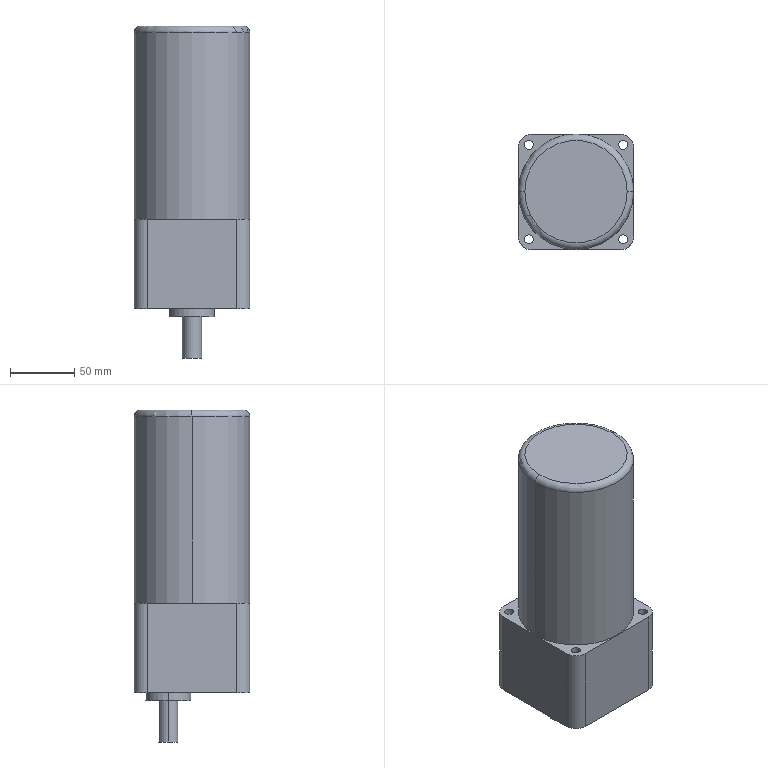Component | SolidWorks | JBM5120-502-01-2-1 | 1 solid | 29 faces | box 90 x 90 x 258.5 mm | volume 1509907 mm3 | cylinder 18 | plane 9 | torus 2 | commonest cylinder face diameters 7 x8 20 x4 15 x2 35 x2 89.8 x2
build123d program:
from build123d import *

# Parameters (mm, degrees)
SKETCH1_W          = 90
SKETCH1_H          = 90
EXTRUDE1_DEPTH     = 69.5
SKETCH2_R          = 44.9
EXTRUDE2_DEPTH     = 150.5
SKETCH3_R          = 3.5
CUT_EXTRUDE1_DEPTH = 230.02
SKETCH4_R          = 17.5
EXTRUDE3_DEPTH     = 6.5
SKETCH5_R          = 7.5
EXTRUDE4_DEPTH     = 32
FILLET1_R          = 10
FILLET2_R          = 5


with BuildPart() as part:
    # Sketch1 → Extrude1 (new body)
    with BuildSketch(Plane.XY):
        Rectangle(SKETCH1_W, SKETCH1_H)
    extrude(amount=-EXTRUDE1_DEPTH)

    # Sketch2 → Extrude2 (add)
    with BuildSketch(Plane(origin=(0, 0, -69.5), x_dir=(-1, 0, 0), z_dir=(0, 0, -1))):
        with Locations(Location((0, 0, 0), (0, 0, 180))):
            Circle(SKETCH2_R)
    extrude(amount=EXTRUDE2_DEPTH)

    # Sketch3 → Cut-Extrude1 (cut, through all)
    with BuildSketch(Plane.XY):
        with Locations((-36.75, 36.75)):
            Circle(SKETCH3_R)
        with Locations((36.75, 36.75)):
            Circle(SKETCH3_R)
        with Locations((36.75, -36.75)):
            Circle(SKETCH3_R)
        with Locations((-36.75, -36.75)):
            Circle(SKETCH3_R)
    extrude(amount=-CUT_EXTRUDE1_DEPTH, mode=Mode.SUBTRACT)

    # Sketch4 → Extrude3 (add)
    with BuildSketch(Plane.XY):
        with Locations(Location((0, 18.5, 0), (0, 0, 180))):
            Circle(SKETCH4_R)
    extrude(amount=EXTRUDE3_DEPTH)

    # Sketch5 → Extrude4 (add)
    with BuildSketch(Plane.XY.offset(6.5)):
        with Locations((0, 18.5)):
            Circle(SKETCH5_R)
    extrude(amount=EXTRUDE4_DEPTH)

    # Fillet1
    fillet1_edges = [part.edges().sort_by_distance(p)[0] for p in [
        (-45, 45, -34.75),
        (45, 45, -34.75),
        (45, -45, -34.75),
        (-45, -45, -34.75),
    ]]
    fillet(fillet1_edges, radius=FILLET1_R)

    # Fillet2
    fillet2_edges = [part.edges().sort_by_distance(p)[0] for p in [
        (-44.9, 0, -220),
    ]]
    fillet(fillet2_edges, radius=FILLET2_R)


solid = part.part

# Placed as in the assembly
solid = solid.moved(Location((647.283, -186.615, -151), (-180, 0, 180)))
STEP:
#1=COLOUR_RGB('',0.7922,0.8196,0.9333);
#2=FILL_AREA_STYLE_COLOUR('',#1);
#3=FILL_AREA_STYLE('',(#2));
#4=SURFACE_STYLE_FILL_AREA(#3);
#5=SURFACE_SIDE_STYLE('',(#4));
#6=SURFACE_STYLE_USAGE(.BOTH.,#5);
#7=PRESENTATION_STYLE_ASSIGNMENT((#6));
#8=CARTESIAN_POINT('',(23.716,-7.347,2.52));
#9=VERTEX_POINT('',#8);
#10=CARTESIAN_POINT('',(27.251,-7.347,2.52));
#11=VERTEX_POINT('',#10);
#12=CARTESIAN_POINT('',(25.484,-7.347,2.52));
#13=DIRECTION('',(0.,0.,-1.));
#14=DIRECTION('',(1.,0.,0.));
#15=AXIS2_PLACEMENT_3D('',#12,#13,#14);
#16=CIRCLE('',#15,1.768);
#17=EDGE_CURVE('',#9,#11,#16,.T.);
#18=ORIENTED_EDGE('',*,*,#17,.F.);
#19=CARTESIAN_POINT('',(23.913,-7.347,2.717));
#20=VERTEX_POINT('',#19);
#21=CARTESIAN_POINT('',(23.913,-7.347,2.52));
#22=DIRECTION('',(0.,1.,0.));
#23=DIRECTION('',(-1.,0.,0.));
#24=AXIS2_PLACEMENT_3D('',#21,#22,#23);
#25=CIRCLE('',#24,0.1969);
#26=EDGE_CURVE('',#9,#20,#25,.T.);
#27=ORIENTED_EDGE('',*,*,#26,.T.);
#28=CARTESIAN_POINT('',(27.054,-7.347,2.717));
#29=VERTEX_POINT('',#28);
#30=CARTESIAN_POINT('',(25.484,-7.347,2.717));
#31=DIRECTION('',(0.,0.,1.));
#32=DIRECTION('',(1.,0.,0.));
#33=AXIS2_PLACEMENT_3D('',#30,#31,#32);
#34=CIRCLE('',#33,1.571);
#35=EDGE_CURVE('',#29,#20,#34,.T.);
#36=ORIENTED_EDGE('',*,*,#35,.F.);
#37=CARTESIAN_POINT('',(27.054,-7.347,2.52));
#38=DIRECTION('',(-0.,-1.,0.));
#39=DIRECTION('',(1.,0.,0.));
#40=AXIS2_PLACEMENT_3D('',#37,#38,#39);
#41=CIRCLE('',#40,0.1969);
#42=EDGE_CURVE('',#11,#29,#41,.T.);
#43=ORIENTED_EDGE('',*,*,#42,.F.);
#44=EDGE_LOOP('',(#18,#27,#36,#43));
#45=FACE_OUTER_BOUND('',#44,.T.);
#46=CARTESIAN_POINT('',(25.484,-7.347,2.52));
#47=DIRECTION('',(0.,0.,1.));
#48=DIRECTION('',(1.,0.,0.));
#49=AXIS2_PLACEMENT_3D('',#46,#47,#48);
#50=TOROIDAL_SURFACE('',#49,1.571,0.1969);
#51=ADVANCED_FACE('',(#45),#50,.T.);
#52=CARTESIAN_POINT('',(25.188,-6.619,-7.461));
#53=VERTEX_POINT('',#52);
#54=CARTESIAN_POINT('',(25.779,-6.619,-7.461));
#55=VERTEX_POINT('',#54);
#56=CARTESIAN_POINT('',(25.484,-6.619,-7.461));
#57=DIRECTION('',(0.,0.,-1.));
#58=DIRECTION('',(-1.,0.,0.));
#59=AXIS2_PLACEMENT_3D('',#56,#57,#58);
#60=CIRCLE('',#59,0.2953);
#61=EDGE_CURVE('',#53,#55,#60,.T.);
#62=ORIENTED_EDGE('',*,*,#61,.F.);
#63=CARTESIAN_POINT('',(25.188,-6.619,-6.201));
#64=VERTEX_POINT('',#63);
#65=CARTESIAN_POINT('',(25.188,-6.619,-7.461));
#66=DIRECTION('',(0.,0.,1.));
#67=VECTOR('',#66,39.37);
#68=LINE('',#65,#67);
#69=EDGE_CURVE('',#53,#64,#68,.T.);
#70=ORIENTED_EDGE('',*,*,#69,.T.);
#71=CARTESIAN_POINT('',(25.779,-6.619,-6.201));
#72=VERTEX_POINT('',#71);
#73=CARTESIAN_POINT('',(25.484,-6.619,-6.201));
#74=DIRECTION('',(0.,0.,-1.));
#75=DIRECTION('',(-1.,0.,0.));
#76=AXIS2_PLACEMENT_3D('',#73,#74,#75);
#77=CIRCLE('',#76,0.2953);
#78=EDGE_CURVE('',#64,#72,#77,.T.);
#79=ORIENTED_EDGE('',*,*,#78,.T.);
#80=CARTESIAN_POINT('',(25.779,-6.619,-7.461));
#81=DIRECTION('',(0.,0.,1.));
#82=VECTOR('',#81,39.37);
#83=LINE('',#80,#82);
#84=EDGE_CURVE('',#55,#72,#83,.T.);
#85=ORIENTED_EDGE('',*,*,#84,.F.);
#86=EDGE_LOOP('',(#62,#70,#79,#85));
#87=FACE_OUTER_BOUND('',#86,.T.);
#88=CARTESIAN_POINT('',(25.484,-6.619,-7.461));
#89=DIRECTION('',(0.,0.,1.));
#90=DIRECTION('',(1.,0.,0.));
#91=AXIS2_PLACEMENT_3D('',#88,#89,#90);
#92=CYLINDRICAL_SURFACE('',#91,0.2953);
#93=ADVANCED_FACE('',(#87),#92,.T.);
#94=CARTESIAN_POINT('',(24.795,-6.619,-6.201));
#95=VERTEX_POINT('',#94);
#96=CARTESIAN_POINT('',(26.173,-6.619,-6.201));
#97=VERTEX_POINT('',#96);
#98=CARTESIAN_POINT('',(25.484,-6.619,-6.201));
#99=DIRECTION('',(0.,0.,-1.));
#100=DIRECTION('',(-1.,0.,0.));
#101=AXIS2_PLACEMENT_3D('',#98,#99,#100);
#102=CIRCLE('',#101,0.689);
#103=EDGE_CURVE('',#95,#97,#102,.T.);
#104=ORIENTED_EDGE('',*,*,#103,.F.);
#105=CARTESIAN_POINT('',(24.795,-6.619,-5.945));
#106=VERTEX_POINT('',#105);
#107=CARTESIAN_POINT('',(24.795,-6.619,-6.201));
#108=DIRECTION('',(0.,0.,1.));
#109=VECTOR('',#108,39.37);
#110=LINE('',#107,#109);
#111=EDGE_CURVE('',#95,#106,#110,.T.);
#112=ORIENTED_EDGE('',*,*,#111,.T.);
#113=CARTESIAN_POINT('',(26.173,-6.619,-5.945));
#114=VERTEX_POINT('',#113);
#115=CARTESIAN_POINT('',(25.484,-6.619,-5.945));
#116=DIRECTION('',(0.,0.,-1.));
#117=DIRECTION('',(-1.,0.,0.));
#118=AXIS2_PLACEMENT_3D('',#115,#116,#117);
#119=CIRCLE('',#118,0.689);
#120=EDGE_CURVE('',#106,#114,#119,.T.);
#121=ORIENTED_EDGE('',*,*,#120,.T.);
#122=CARTESIAN_POINT('',(26.173,-6.619,-6.201));
#123=DIRECTION('',(0.,0.,1.));
#124=VECTOR('',#123,39.37);
#125=LINE('',#122,#124);
#126=EDGE_CURVE('',#97,#114,#125,.T.);
#127=ORIENTED_EDGE('',*,*,#126,.F.);
#128=EDGE_LOOP('',(#104,#112,#121,#127));
#129=FACE_OUTER_BOUND('',#128,.T.);
#130=CARTESIAN_POINT('',(25.484,-6.619,-6.201));
#131=DIRECTION('',(0.,0.,1.));
#132=DIRECTION('',(1.,0.,0.));
#133=AXIS2_PLACEMENT_3D('',#130,#131,#132);
#134=CYLINDRICAL_SURFACE('',#133,0.689);
#135=ADVANCED_FACE('',(#129),#134,.T.);
#136=CARTESIAN_POINT('',(27.068,-8.794,-3.209));
#137=VERTEX_POINT('',#136);
#138=CARTESIAN_POINT('',(26.793,-8.794,-3.209));
#139=VERTEX_POINT('',#138);
#140=CARTESIAN_POINT('',(26.93,-8.794,-3.209));
#141=DIRECTION('',(0.,0.,-1.));
#142=DIRECTION('',(-1.,0.,0.));
#143=AXIS2_PLACEMENT_3D('',#140,#141,#142);
#144=CIRCLE('',#143,0.1378);
#145=EDGE_CURVE('',#137,#139,#144,.T.);
#146=ORIENTED_EDGE('',*,*,#145,.F.);
#147=CARTESIAN_POINT('',(27.068,-8.794,-5.945));
#148=VERTEX_POINT('',#147);
#149=CARTESIAN_POINT('',(27.068,-8.794,2.717));
#150=DIRECTION('',(0.,0.,-1.));
#151=VECTOR('',#150,39.37);
#152=LINE('',#149,#151);
#153=EDGE_CURVE('',#137,#148,#152,.T.);
#154=ORIENTED_EDGE('',*,*,#153,.T.);
#155=CARTESIAN_POINT('',(26.793,-8.794,-5.945));
#156=VERTEX_POINT('',#155);
#157=CARTESIAN_POINT('',(26.93,-8.794,-5.945));
#158=DIRECTION('',(0.,0.,-1.));
#159=DIRECTION('',(1.,0.,0.));
#160=AXIS2_PLACEMENT_3D('',#157,#158,#159);
#161=CIRCLE('',#160,0.1378);
#162=EDGE_CURVE('',#148,#156,#161,.T.);
#163=ORIENTED_EDGE('',*,*,#162,.T.);
#164=CARTESIAN_POINT('',(26.793,-8.794,2.717));
#165=DIRECTION('',(0.,0.,-1.));
#166=VECTOR('',#165,39.37);
#167=LINE('',#164,#166);
#168=EDGE_CURVE('',#139,#156,#167,.T.);
#169=ORIENTED_EDGE('',*,*,#168,.F.);
#170=EDGE_LOOP('',(#146,#154,#163,#169));
#171=FACE_OUTER_BOUND('',#170,.T.);
#172=CARTESIAN_POINT('',(26.93,-8.794,2.717));
#173=DIRECTION('',(0.,0.,-1.));
#174=DIRECTION('',(-1.,0.,0.));
#175=AXIS2_PLACEMENT_3D('',#172,#173,#174);
#176=CYLINDRICAL_SURFACE('',#175,0.1378);
#177=ADVANCED_FACE('',(#171),#176,.F.);
#178=CARTESIAN_POINT('',(24.175,-8.794,-3.209));
#179=VERTEX_POINT('',#178);
#180=CARTESIAN_POINT('',(23.899,-8.794,-3.209));
#181=VERTEX_POINT('',#180);
#182=CARTESIAN_POINT('',(24.037,-8.794,-3.209));
#183=DIRECTION('',(0.,0.,-1.));
#184=DIRECTION('',(-1.,0.,0.));
#185=AXIS2_PLACEMENT_3D('',#182,#183,#184);
#186=CIRCLE('',#185,0.1378);
#187=EDGE_CURVE('',#179,#181,#186,.T.);
#188=ORIENTED_EDGE('',*,*,#187,.F.);
#189=CARTESIAN_POINT('',(24.175,-8.794,-5.945));
#190=VERTEX_POINT('',#189);
#191=CARTESIAN_POINT('',(24.175,-8.794,2.717));
#192=DIRECTION('',(0.,0.,-1.));
#193=VECTOR('',#192,39.37);
#194=LINE('',#191,#193);
#195=EDGE_CURVE('',#179,#190,#194,.T.);
#196=ORIENTED_EDGE('',*,*,#195,.T.);
#197=CARTESIAN_POINT('',(23.899,-8.794,-5.945));
#198=VERTEX_POINT('',#197);
#199=CARTESIAN_POINT('',(24.037,-8.794,-5.945));
#200=DIRECTION('',(0.,0.,-1.));
#201=DIRECTION('',(-1.,0.,0.));
#202=AXIS2_PLACEMENT_3D('',#199,#200,#201);
#203=CIRCLE('',#202,0.1378);
#204=EDGE_CURVE('',#190,#198,#203,.T.);
#205=ORIENTED_EDGE('',*,*,#204,.T.);
#206=CARTESIAN_POINT('',(23.899,-8.794,2.717));
#207=DIRECTION('',(0.,0.,-1.));
#208=VECTOR('',#207,39.37);
#209=LINE('',#206,#208);
#210=EDGE_CURVE('',#181,#198,#209,.T.);
#211=ORIENTED_EDGE('',*,*,#210,.F.);
#212=EDGE_LOOP('',(#188,#196,#205,#211));
#213=FACE_OUTER_BOUND('',#212,.T.);
#214=CARTESIAN_POINT('',(24.037,-8.794,2.717));
#215=DIRECTION('',(0.,0.,-1.));
#216=DIRECTION('',(-1.,0.,0.));
#217=AXIS2_PLACEMENT_3D('',#214,#215,#216);
#218=CYLINDRICAL_SURFACE('',#217,0.1378);
#219=ADVANCED_FACE('',(#213),#218,.F.);
#220=CARTESIAN_POINT('',(24.175,-5.9,-3.209));
#221=VERTEX_POINT('',#220);
#222=CARTESIAN_POINT('',(23.899,-5.9,-3.209));
#223=VERTEX_POINT('',#222);
#224=CARTESIAN_POINT('',(24.037,-5.9,-3.209));
#225=DIRECTION('',(0.,0.,-1.));
#226=DIRECTION('',(-1.,0.,0.));
#227=AXIS2_PLACEMENT_3D('',#224,#225,#226);
#228=CIRCLE('',#227,0.1378);
#229=EDGE_CURVE('',#221,#223,#228,.T.);
#230=ORIENTED_EDGE('',*,*,#229,.F.);
#231=CARTESIAN_POINT('',(24.175,-5.9,-5.945));
#232=VERTEX_POINT('',#231);
#233=CARTESIAN_POINT('',(24.175,-5.9,2.717));
#234=DIRECTION('',(0.,0.,-1.));
#235=VECTOR('',#234,39.37);
#236=LINE('',#233,#235);
#237=EDGE_CURVE('',#221,#232,#236,.T.);
#238=ORIENTED_EDGE('',*,*,#237,.T.);
#239=CARTESIAN_POINT('',(23.899,-5.9,-5.945));
#240=VERTEX_POINT('',#239);
#241=CARTESIAN_POINT('',(24.037,-5.9,-5.945));
#242=DIRECTION('',(0.,0.,-1.));
#243=DIRECTION('',(1.,0.,0.));
#244=AXIS2_PLACEMENT_3D('',#241,#242,#243);
#245=CIRCLE('',#244,0.1378);
#246=EDGE_CURVE('',#232,#240,#245,.T.);
#247=ORIENTED_EDGE('',*,*,#246,.T.);
#248=CARTESIAN_POINT('',(23.899,-5.9,2.717));
#249=DIRECTION('',(0.,0.,-1.));
#250=VECTOR('',#249,39.37);
#251=LINE('',#248,#250);
#252=EDGE_CURVE('',#223,#240,#251,.T.);
#253=ORIENTED_EDGE('',*,*,#252,.F.);
#254=EDGE_LOOP('',(#230,#238,#247,#253));
#255=FACE_OUTER_BOUND('',#254,.T.);
#256=CARTESIAN_POINT('',(24.037,-5.9,2.717));
#257=DIRECTION('',(0.,0.,-1.));
#258=DIRECTION('',(-1.,0.,0.));
#259=AXIS2_PLACEMENT_3D('',#256,#257,#258);
#260=CYLINDRICAL_SURFACE('',#259,0.1378);
#261=ADVANCED_FACE('',(#255),#260,.F.);
#262=CARTESIAN_POINT('',(27.068,-5.9,-3.209));
#263=VERTEX_POINT('',#262);
#264=CARTESIAN_POINT('',(26.793,-5.9,-3.209));
#265=VERTEX_POINT('',#264);
#266=CARTESIAN_POINT('',(26.93,-5.9,-3.209));
#267=DIRECTION('',(0.,0.,-1.));
#268=DIRECTION('',(-1.,0.,0.));
#269=AXIS2_PLACEMENT_3D('',#266,#267,#268);
#270=CIRCLE('',#269,0.1378);
#271=EDGE_CURVE('',#263,#265,#270,.T.);
#272=ORIENTED_EDGE('',*,*,#271,.F.);
#273=CARTESIAN_POINT('',(27.068,-5.9,-5.945));
#274=VERTEX_POINT('',#273);
#275=CARTESIAN_POINT('',(27.068,-5.9,2.717));
#276=DIRECTION('',(0.,0.,-1.));
#277=VECTOR('',#276,39.37);
#278=LINE('',#275,#277);
#279=EDGE_CURVE('',#263,#274,#278,.T.);
#280=ORIENTED_EDGE('',*,*,#279,.T.);
#281=CARTESIAN_POINT('',(26.793,-5.9,-5.945));
#282=VERTEX_POINT('',#281);
#283=CARTESIAN_POINT('',(26.93,-5.9,-5.945));
#284=DIRECTION('',(0.,0.,-1.));
#285=DIRECTION('',(-1.,0.,0.));
#286=AXIS2_PLACEMENT_3D('',#283,#284,#285);
#287=CIRCLE('',#286,0.1378);
#288=EDGE_CURVE('',#274,#282,#287,.T.);
#289=ORIENTED_EDGE('',*,*,#288,.T.);
#290=CARTESIAN_POINT('',(26.793,-5.9,2.717));
#291=DIRECTION('',(0.,0.,-1.));
#292=VECTOR('',#291,39.37);
#293=LINE('',#290,#292);
#294=EDGE_CURVE('',#265,#282,#293,.T.);
#295=ORIENTED_EDGE('',*,*,#294,.F.);
#296=EDGE_LOOP('',(#272,#280,#289,#295));
#297=FACE_OUTER_BOUND('',#296,.T.);
#298=CARTESIAN_POINT('',(26.93,-5.9,2.717));
#299=DIRECTION('',(0.,0.,-1.));
#300=DIRECTION('',(-1.,0.,0.));
#301=AXIS2_PLACEMENT_3D('',#298,#299,#300);
#302=CYLINDRICAL_SURFACE('',#301,0.1378);
#303=ADVANCED_FACE('',(#297),#302,.F.);
#304=ORIENTED_EDGE('',*,*,#17,.T.);
#305=CARTESIAN_POINT('',(27.251,-7.347,-3.209));
#306=VERTEX_POINT('',#305);
#307=CARTESIAN_POINT('',(27.251,-7.347,2.717));
#308=DIRECTION('',(0.,0.,-1.));
#309=VECTOR('',#308,39.37);
#310=LINE('',#307,#309);
#311=EDGE_CURVE('',#11,#306,#310,.T.);
#312=ORIENTED_EDGE('',*,*,#311,.T.);
#313=CARTESIAN_POINT('',(23.716,-7.347,-3.209));
#314=VERTEX_POINT('',#313);
#315=CARTESIAN_POINT('',(25.484,-7.347,-3.209));
#316=DIRECTION('',(0.,0.,1.));
#317=DIRECTION('',(-1.,0.,0.));
#318=AXIS2_PLACEMENT_3D('',#315,#316,#317);
#319=CIRCLE('',#318,1.768);
#320=EDGE_CURVE('',#306,#314,#319,.T.);
#321=ORIENTED_EDGE('',*,*,#320,.T.);
#322=CARTESIAN_POINT('',(23.716,-7.347,2.717));
#323=DIRECTION('',(0.,0.,-1.));
#324=VECTOR('',#323,39.37);
#325=LINE('',#322,#324);
#326=EDGE_CURVE('',#9,#314,#325,.T.);
#327=ORIENTED_EDGE('',*,*,#326,.F.);
#328=EDGE_LOOP('',(#304,#312,#321,#327));
#329=FACE_OUTER_BOUND('',#328,.T.);
#330=CARTESIAN_POINT('',(25.484,-7.347,2.717));
#331=DIRECTION('',(0.,0.,-1.));
#332=DIRECTION('',(-1.,0.,0.));
#333=AXIS2_PLACEMENT_3D('',#330,#331,#332);
#334=CYLINDRICAL_SURFACE('',#333,1.768);
#335=ADVANCED_FACE('',(#329),#334,.T.);
#336=CARTESIAN_POINT('',(25.484,-6.619,-6.201));
#337=DIRECTION('',(0.,0.,-1.));
#338=DIRECTION('',(-1.,0.,0.));
#339=AXIS2_PLACEMENT_3D('',#336,#337,#338);
#340=CIRCLE('',#339,0.689);
#341=EDGE_CURVE('',#97,#95,#340,.T.);
#342=ORIENTED_EDGE('',*,*,#341,.T.);
#343=ORIENTED_EDGE('',*,*,#103,.T.);
#344=EDGE_LOOP('',(#342,#343));
#345=FACE_OUTER_BOUND('',#344,.T.);
#346=CARTESIAN_POINT('',(25.484,-6.619,-6.201));
#347=DIRECTION('',(0.,0.,-1.));
#348=DIRECTION('',(-1.,0.,0.));
#349=AXIS2_PLACEMENT_3D('',#346,#347,#348);
#350=CIRCLE('',#349,0.2953);
#351=EDGE_CURVE('',#72,#64,#350,.T.);
#352=ORIENTED_EDGE('',*,*,#351,.F.);
#353=ORIENTED_EDGE('',*,*,#78,.F.);
#354=EDGE_LOOP('',(#352,#353));
#355=FACE_BOUND('',#354,.T.);
#356=CARTESIAN_POINT('',(25.484,-6.619,-6.201));
#357=DIRECTION('',(0.,0.,-1.));
#358=DIRECTION('',(-1.,0.,0.));
#359=AXIS2_PLACEMENT_3D('',#356,#357,#358);
#360=PLANE('',#359);
#361=ADVANCED_FACE('',(#345,#355),#360,.T.);
#362=CARTESIAN_POINT('',(27.255,-5.969,-5.945));
#363=VERTEX_POINT('',#362);
#364=CARTESIAN_POINT('',(27.255,-8.725,-5.945));
#365=VERTEX_POINT('',#364);
#366=CARTESIAN_POINT('',(27.255,-5.575,-5.945));
#367=DIRECTION('',(-0.,-1.,0.));
#368=VECTOR('',#367,39.37);
#369=LINE('',#366,#368);
#370=EDGE_CURVE('',#363,#365,#369,.T.);
#371=ORIENTED_EDGE('',*,*,#370,.T.);
#372=CARTESIAN_POINT('',(26.862,-9.119,-5.945));
#373=VERTEX_POINT('',#372);
#374=CARTESIAN_POINT('',(26.862,-8.725,-5.945));
#375=DIRECTION('',(0.,0.,-1.));
#376=DIRECTION('',(-1.,0.,0.));
#377=AXIS2_PLACEMENT_3D('',#374,#375,#376);
#378=CIRCLE('',#377,0.3937);
#379=EDGE_CURVE('',#365,#373,#378,.T.);
#380=ORIENTED_EDGE('',*,*,#379,.T.);
#381=CARTESIAN_POINT('',(24.106,-9.119,-5.945));
#382=VERTEX_POINT('',#381);
#383=CARTESIAN_POINT('',(27.255,-9.119,-5.945));
#384=DIRECTION('',(-1.,0.,0.));
#385=VECTOR('',#384,39.37);
#386=LINE('',#383,#385);
#387=EDGE_CURVE('',#373,#382,#386,.T.);
#388=ORIENTED_EDGE('',*,*,#387,.T.);
#389=CARTESIAN_POINT('',(23.712,-8.725,-5.945));
#390=VERTEX_POINT('',#389);
#391=CARTESIAN_POINT('',(24.106,-8.725,-5.945));
#392=DIRECTION('',(0.,0.,-1.));
#393=DIRECTION('',(-1.,0.,0.));
#394=AXIS2_PLACEMENT_3D('',#391,#392,#393);
#395=CIRCLE('',#394,0.3937);
#396=EDGE_CURVE('',#382,#390,#395,.T.);
#397=ORIENTED_EDGE('',*,*,#396,.T.);
#398=CARTESIAN_POINT('',(23.712,-5.969,-5.945));
#399=VERTEX_POINT('',#398);
#400=CARTESIAN_POINT('',(23.712,-5.575,-5.945));
#401=DIRECTION('',(0.,1.,0.));
#402=VECTOR('',#401,39.37);
#403=LINE('',#400,#402);
#404=EDGE_CURVE('',#390,#399,#403,.T.);
#405=ORIENTED_EDGE('',*,*,#404,.T.);
#406=CARTESIAN_POINT('',(24.106,-5.575,-5.945));
#407=VERTEX_POINT('',#406);
#408=CARTESIAN_POINT('',(24.106,-5.969,-5.945));
#409=DIRECTION('',(0.,0.,-1.));
#410=DIRECTION('',(-1.,0.,0.));
#411=AXIS2_PLACEMENT_3D('',#408,#409,#410);
#412=CIRCLE('',#411,0.3937);
#413=EDGE_CURVE('',#399,#407,#412,.T.);
#414=ORIENTED_EDGE('',*,*,#413,.T.);
#415=CARTESIAN_POINT('',(26.862,-5.575,-5.945));
#416=VERTEX_POINT('',#415);
#417=CARTESIAN_POINT('',(27.255,-5.575,-5.945));
#418=DIRECTION('',(1.,-0.,0.));
#419=VECTOR('',#418,39.37);
#420=LINE('',#417,#419);
#421=EDGE_CURVE('',#407,#416,#420,.T.);
#422=ORIENTED_EDGE('',*,*,#421,.T.);
#423=CARTESIAN_POINT('',(26.862,-5.969,-5.945));
#424=DIRECTION('',(0.,0.,-1.));
#425=DIRECTION('',(-1.,0.,0.));
#426=AXIS2_PLACEMENT_3D('',#423,#424,#425);
#427=CIRCLE('',#426,0.3937);
#428=EDGE_CURVE('',#416,#363,#427,.T.);
#429=ORIENTED_EDGE('',*,*,#428,.T.);
#430=EDGE_LOOP('',(#371,#380,#388,#397,#405,#414,#422,#429));
#431=FACE_OUTER_BOUND('',#430,.T.);
#432=CARTESIAN_POINT('',(26.93,-5.9,-5.945));
#433=DIRECTION('',(0.,0.,-1.));
#434=DIRECTION('',(-1.,0.,0.));
#435=AXIS2_PLACEMENT_3D('',#432,#433,#434);
#436=CIRCLE('',#435,0.1378);
#437=EDGE_CURVE('',#282,#274,#436,.T.);
#438=ORIENTED_EDGE('',*,*,#437,.F.);
#439=ORIENTED_EDGE('',*,*,#288,.F.);
#440=EDGE_LOOP('',(#438,#439));
#441=FACE_BOUND('',#440,.T.);
#442=CARTESIAN_POINT('',(24.037,-5.9,-5.945));
#443=DIRECTION('',(0.,0.,-1.));
#444=DIRECTION('',(1.,0.,0.));
#445=AXIS2_PLACEMENT_3D('',#442,#443,#444);
#446=CIRCLE('',#445,0.1378);
#447=EDGE_CURVE('',#240,#232,#446,.T.);
#448=ORIENTED_EDGE('',*,*,#447,.F.);
#449=ORIENTED_EDGE('',*,*,#246,.F.);
#450=EDGE_LOOP('',(#448,#449));
#451=FACE_BOUND('',#450,.T.);
#452=CARTESIAN_POINT('',(24.037,-8.794,-5.945));
#453=DIRECTION('',(0.,0.,-1.));
#454=DIRECTION('',(-1.,0.,0.));
#455=AXIS2_PLACEMENT_3D('',#452,#453,#454);
#456=CIRCLE('',#455,0.1378);
#457=EDGE_CURVE('',#198,#190,#456,.T.);
#458=ORIENTED_EDGE('',*,*,#457,.F.);
#459=ORIENTED_EDGE('',*,*,#204,.F.);
#460=EDGE_LOOP('',(#458,#459));
#461=FACE_BOUND('',#460,.T.);
#462=CARTESIAN_POINT('',(26.93,-8.794,-5.945));
#463=DIRECTION('',(0.,0.,-1.));
#464=DIRECTION('',(1.,0.,0.));
#465=AXIS2_PLACEMENT_3D('',#462,#463,#464);
#466=CIRCLE('',#465,0.1378);
#467=EDGE_CURVE('',#156,#148,#466,.T.);
#468=ORIENTED_EDGE('',*,*,#467,.F.);
#469=ORIENTED_EDGE('',*,*,#162,.F.);
#470=EDGE_LOOP('',(#468,#469));
#471=FACE_BOUND('',#470,.T.);
#472=CARTESIAN_POINT('',(25.484,-6.619,-5.945));
#473=DIRECTION('',(0.,0.,-1.));
#474=DIRECTION('',(-1.,0.,0.));
#475=AXIS2_PLACEMENT_3D('',#472,#473,#474);
#476=CIRCLE('',#475,0.689);
#477=EDGE_CURVE('',#114,#106,#476,.T.);
#478=ORIENTED_EDGE('',*,*,#477,.F.);
#479=ORIENTED_EDGE('',*,*,#120,.F.);
#480=EDGE_LOOP('',(#478,#479));
#481=FACE_BOUND('',#480,.T.);
#482=CARTESIAN_POINT('',(27.255,-9.119,-5.945));
#483=DIRECTION('',(0.,0.,-1.));
#484=DIRECTION('',(-1.,0.,0.));
#485=AXIS2_PLACEMENT_3D('',#482,#483,#484);
#486=PLANE('',#485);
#487=ADVANCED_FACE('',(#431,#441,#451,#461,#471,#481),#486,.T.);
#488=CARTESIAN_POINT('',(26.93,-8.794,-3.209));
#489=DIRECTION('',(0.,0.,-1.));
#490=DIRECTION('',(-1.,0.,0.));
#491=AXIS2_PLACEMENT_3D('',#488,#489,#490);
#492=CIRCLE('',#491,0.1378);
#493=EDGE_CURVE('',#139,#137,#492,.T.);
#494=ORIENTED_EDGE('',*,*,#493,.T.);
#495=ORIENTED_EDGE('',*,*,#145,.T.);
#496=EDGE_LOOP('',(#494,#495));
#497=FACE_BOUND('',#496,.T.);
#498=CARTESIAN_POINT('',(24.037,-8.794,-3.209));
#499=DIRECTION('',(0.,0.,-1.));
#500=DIRECTION('',(-1.,0.,0.));
#501=AXIS2_PLACEMENT_3D('',#498,#499,#500);
#502=CIRCLE('',#501,0.1378);
#503=EDGE_CURVE('',#181,#179,#502,.T.);
#504=ORIENTED_EDGE('',*,*,#503,.T.);
#505=ORIENTED_EDGE('',*,*,#187,.T.);
#506=EDGE_LOOP('',(#504,#505));
#507=FACE_BOUND('',#506,.T.);
#508=CARTESIAN_POINT('',(24.037,-5.9,-3.209));
#509=DIRECTION('',(0.,0.,-1.));
#510=DIRECTION('',(-1.,0.,0.));
#511=AXIS2_PLACEMENT_3D('',#508,#509,#510);
#512=CIRCLE('',#511,0.1378);
#513=EDGE_CURVE('',#223,#221,#512,.T.);
#514=ORIENTED_EDGE('',*,*,#513,.T.);
#515=ORIENTED_EDGE('',*,*,#229,.T.);
#516=EDGE_LOOP('',(#514,#515));
#517=FACE_BOUND('',#516,.T.);
#518=CARTESIAN_POINT('',(26.93,-5.9,-3.209));
#519=DIRECTION('',(0.,0.,-1.));
#520=DIRECTION('',(-1.,0.,0.));
#521=AXIS2_PLACEMENT_3D('',#518,#519,#520);
#522=CIRCLE('',#521,0.1378);
#523=EDGE_CURVE('',#265,#263,#522,.T.);
#524=ORIENTED_EDGE('',*,*,#523,.T.);
#525=ORIENTED_EDGE('',*,*,#271,.T.);
#526=EDGE_LOOP('',(#524,#525));
#527=FACE_BOUND('',#526,.T.);
#528=CARTESIAN_POINT('',(26.862,-9.119,-3.209));
#529=VERTEX_POINT('',#528);
#530=CARTESIAN_POINT('',(24.106,-9.119,-3.209));
#531=VERTEX_POINT('',#530);
#532=CARTESIAN_POINT('',(27.255,-9.119,-3.209));
#533=DIRECTION('',(-1.,0.,0.));
#534=VECTOR('',#533,39.37);
#535=LINE('',#532,#534);
#536=EDGE_CURVE('',#529,#531,#535,.T.);
#537=ORIENTED_EDGE('',*,*,#536,.F.);
#538=CARTESIAN_POINT('',(27.255,-8.725,-3.209));
#539=VERTEX_POINT('',#538);
#540=CARTESIAN_POINT('',(26.862,-8.725,-3.209));
#541=DIRECTION('',(0.,0.,1.));
#542=DIRECTION('',(-1.,0.,0.));
#543=AXIS2_PLACEMENT_3D('',#540,#541,#542);
#544=CIRCLE('',#543,0.3937);
#545=EDGE_CURVE('',#529,#539,#544,.T.);
#546=ORIENTED_EDGE('',*,*,#545,.T.);
#547=CARTESIAN_POINT('',(27.255,-5.969,-3.209));
#548=VERTEX_POINT('',#547);
#549=CARTESIAN_POINT('',(27.255,-5.575,-3.209));
#550=DIRECTION('',(-0.,-1.,0.));
#551=VECTOR('',#550,39.37);
#552=LINE('',#549,#551);
#553=EDGE_CURVE('',#548,#539,#552,.T.);
#554=ORIENTED_EDGE('',*,*,#553,.F.);
#555=CARTESIAN_POINT('',(26.862,-5.575,-3.209));
#556=VERTEX_POINT('',#555);
#557=CARTESIAN_POINT('',(26.862,-5.969,-3.209));
#558=DIRECTION('',(0.,0.,1.));
#559=DIRECTION('',(-1.,0.,0.));
#560=AXIS2_PLACEMENT_3D('',#557,#558,#559);
#561=CIRCLE('',#560,0.3937);
#562=EDGE_CURVE('',#548,#556,#561,.T.);
#563=ORIENTED_EDGE('',*,*,#562,.T.);
#564=CARTESIAN_POINT('',(24.106,-5.575,-3.209));
#565=VERTEX_POINT('',#564);
#566=CARTESIAN_POINT('',(27.255,-5.575,-3.209));
#567=DIRECTION('',(1.,-0.,0.));
#568=VECTOR('',#567,39.37);
#569=LINE('',#566,#568);
#570=EDGE_CURVE('',#565,#556,#569,.T.);
#571=ORIENTED_EDGE('',*,*,#570,.F.);
#572=CARTESIAN_POINT('',(23.712,-5.969,-3.209));
#573=VERTEX_POINT('',#572);
#574=CARTESIAN_POINT('',(24.106,-5.969,-3.209));
#575=DIRECTION('',(0.,0.,1.));
#576=DIRECTION('',(-1.,-0.,0.));
#577=AXIS2_PLACEMENT_3D('',#574,#575,#576);
#578=CIRCLE('',#577,0.3937);
#579=EDGE_CURVE('',#565,#573,#578,.T.);
#580=ORIENTED_EDGE('',*,*,#579,.T.);
#581=CARTESIAN_POINT('',(23.712,-8.725,-3.209));
#582=VERTEX_POINT('',#581);
#583=CARTESIAN_POINT('',(23.712,-5.575,-3.209));
#584=DIRECTION('',(0.,1.,0.));
#585=VECTOR('',#584,39.37);
#586=LINE('',#583,#585);
#587=EDGE_CURVE('',#582,#573,#586,.T.);
#588=ORIENTED_EDGE('',*,*,#587,.F.);
#589=CARTESIAN_POINT('',(24.106,-8.725,-3.209));
#590=DIRECTION('',(0.,0.,1.));
#591=DIRECTION('',(-1.,0.,0.));
#592=AXIS2_PLACEMENT_3D('',#589,#590,#591);
#593=CIRCLE('',#592,0.3937);
#594=EDGE_CURVE('',#582,#531,#593,.T.);
#595=ORIENTED_EDGE('',*,*,#594,.T.);
#596=EDGE_LOOP('',(#537,#546,#554,#563,#571,#580,#588,#595));
#597=FACE_OUTER_BOUND('',#596,.T.);
#598=CARTESIAN_POINT('',(25.484,-7.347,-3.209));
#599=DIRECTION('',(0.,0.,1.));
#600=DIRECTION('',(-1.,0.,0.));
#601=AXIS2_PLACEMENT_3D('',#598,#599,#600);
#602=CIRCLE('',#601,1.768);
#603=EDGE_CURVE('',#314,#306,#602,.T.);
#604=ORIENTED_EDGE('',*,*,#603,.F.);
#605=ORIENTED_EDGE('',*,*,#320,.F.);
#606=EDGE_LOOP('',(#604,#605));
#607=FACE_BOUND('',#606,.T.);
#608=CARTESIAN_POINT('',(27.255,-9.119,-3.209));
#609=DIRECTION('',(0.,0.,-1.));
#610=DIRECTION('',(-1.,0.,0.));
#611=AXIS2_PLACEMENT_3D('',#608,#609,#610);
#612=PLANE('',#611);
#613=ADVANCED_FACE('',(#497,#507,#517,#527,#597,#607),#612,.F.);
#614=ORIENTED_EDGE('',*,*,#553,.T.);
#615=CARTESIAN_POINT('',(27.255,-8.725,-3.209));
#616=DIRECTION('',(0.,0.,-1.));
#617=VECTOR('',#616,39.37);
#618=LINE('',#615,#617);
#619=EDGE_CURVE('',#539,#365,#618,.T.);
#620=ORIENTED_EDGE('',*,*,#619,.T.);
#621=ORIENTED_EDGE('',*,*,#370,.F.);
#622=CARTESIAN_POINT('',(27.255,-5.969,-3.209));
#623=DIRECTION('',(0.,0.,1.));
#624=VECTOR('',#623,39.37);
#625=LINE('',#622,#624);
#626=EDGE_CURVE('',#363,#548,#625,.T.);
#627=ORIENTED_EDGE('',*,*,#626,.T.);
#628=EDGE_LOOP('',(#614,#620,#621,#627));
#629=FACE_OUTER_BOUND('',#628,.T.);
#630=CARTESIAN_POINT('',(27.255,-5.575,-3.209));
#631=DIRECTION('',(1.,-0.,0.));
#632=DIRECTION('',(-0.,-1.,0.));
#633=AXIS2_PLACEMENT_3D('',#630,#631,#632);
#634=PLANE('',#633);
#635=ADVANCED_FACE('',(#629),#634,.T.);
#636=ORIENTED_EDGE('',*,*,#570,.T.);
#637=CARTESIAN_POINT('',(26.862,-5.575,-3.209));
#638=DIRECTION('',(0.,0.,-1.));
#639=VECTOR('',#638,39.37);
#640=LINE('',#637,#639);
#641=EDGE_CURVE('',#556,#416,#640,.T.);
#642=ORIENTED_EDGE('',*,*,#641,.T.);
#643=ORIENTED_EDGE('',*,*,#421,.F.);
#644=CARTESIAN_POINT('',(24.106,-5.575,-3.209));
#645=DIRECTION('',(0.,0.,1.));
#646=VECTOR('',#645,39.37);
#647=LINE('',#644,#646);
#648=EDGE_CURVE('',#407,#565,#647,.T.);
#649=ORIENTED_EDGE('',*,*,#648,.T.);
#650=EDGE_LOOP('',(#636,#642,#643,#649));
#651=FACE_OUTER_BOUND('',#650,.T.);
#652=CARTESIAN_POINT('',(27.255,-5.575,-3.209));
#653=DIRECTION('',(0.,1.,0.));
#654=DIRECTION('',(1.,-0.,0.));
#655=AXIS2_PLACEMENT_3D('',#652,#653,#654);
#656=PLANE('',#655);
#657=ADVANCED_FACE('',(#651),#656,.T.);
#658=ORIENTED_EDGE('',*,*,#404,.F.);
#659=CARTESIAN_POINT('',(23.712,-8.725,-3.209));
#660=DIRECTION('',(0.,0.,1.));
#661=VECTOR('',#660,39.37);
#662=LINE('',#659,#661);
#663=EDGE_CURVE('',#390,#582,#662,.T.);
#664=ORIENTED_EDGE('',*,*,#663,.T.);
#665=ORIENTED_EDGE('',*,*,#587,.T.);
#666=CARTESIAN_POINT('',(23.712,-5.969,-3.209));
#667=DIRECTION('',(0.,0.,-1.));
#668=VECTOR('',#667,39.37);
#669=LINE('',#666,#668);
#670=EDGE_CURVE('',#573,#399,#669,.T.);
#671=ORIENTED_EDGE('',*,*,#670,.T.);
#672=EDGE_LOOP('',(#658,#664,#665,#671));
#673=FACE_OUTER_BOUND('',#672,.T.);
#674=CARTESIAN_POINT('',(23.712,-5.575,-3.209));
#675=DIRECTION('',(-1.,0.,0.));
#676=DIRECTION('',(0.,1.,0.));
#677=AXIS2_PLACEMENT_3D('',#674,#675,#676);
#678=PLANE('',#677);
#679=ADVANCED_FACE('',(#673),#678,.T.);
#680=ORIENTED_EDGE('',*,*,#387,.F.);
#681=CARTESIAN_POINT('',(26.862,-9.119,-3.209));
#682=DIRECTION('',(0.,0.,1.));
#683=VECTOR('',#682,39.37);
#684=LINE('',#681,#683);
#685=EDGE_CURVE('',#373,#529,#684,.T.);
#686=ORIENTED_EDGE('',*,*,#685,.T.);
#687=ORIENTED_EDGE('',*,*,#536,.T.);
#688=CARTESIAN_POINT('',(24.106,-9.119,-3.209));
#689=DIRECTION('',(0.,0.,-1.));
#690=VECTOR('',#689,39.37);
#691=LINE('',#688,#690);
#692=EDGE_CURVE('',#531,#382,#691,.T.);
#693=ORIENTED_EDGE('',*,*,#692,.T.);
#694=EDGE_LOOP('',(#680,#686,#687,#693));
#695=FACE_OUTER_BOUND('',#694,.T.);
#696=CARTESIAN_POINT('',(27.255,-9.119,-3.209));
#697=DIRECTION('',(-0.,-1.,0.));
#698=DIRECTION('',(-1.,0.,0.));
#699=AXIS2_PLACEMENT_3D('',#696,#697,#698);
#700=PLANE('',#699);
#701=ADVANCED_FACE('',(#695),#700,.T.);
#702=ORIENTED_EDGE('',*,*,#311,.F.);
#703=CARTESIAN_POINT('',(25.484,-7.347,2.52));
#704=DIRECTION('',(0.,0.,-1.));
#705=DIRECTION('',(1.,0.,0.));
#706=AXIS2_PLACEMENT_3D('',#703,#704,#705);
#707=CIRCLE('',#706,1.768);
#708=EDGE_CURVE('',#11,#9,#707,.T.);
#709=ORIENTED_EDGE('',*,*,#708,.T.);
#710=ORIENTED_EDGE('',*,*,#326,.T.);
#711=ORIENTED_EDGE('',*,*,#603,.T.);
#712=EDGE_LOOP('',(#702,#709,#710,#711));
#713=FACE_OUTER_BOUND('',#712,.T.);
#714=CARTESIAN_POINT('',(25.484,-7.347,2.717));
#715=DIRECTION('',(0.,0.,-1.));
#716=DIRECTION('',(-1.,0.,0.));
#717=AXIS2_PLACEMENT_3D('',#714,#715,#716);
#718=CYLINDRICAL_SURFACE('',#717,1.768);
#719=ADVANCED_FACE('',(#713),#718,.T.);
#720=ORIENTED_EDGE('',*,*,#35,.T.);
#721=CARTESIAN_POINT('',(25.484,-7.347,2.717));
#722=DIRECTION('',(0.,0.,1.));
#723=DIRECTION('',(1.,0.,0.));
#724=AXIS2_PLACEMENT_3D('',#721,#722,#723);
#725=CIRCLE('',#724,1.571);
#726=EDGE_CURVE('',#20,#29,#725,.T.);
#727=ORIENTED_EDGE('',*,*,#726,.T.);
#728=EDGE_LOOP('',(#720,#727));
#729=FACE_OUTER_BOUND('',#728,.T.);
#730=CARTESIAN_POINT('',(25.484,-7.347,2.717));
#731=DIRECTION('',(0.,0.,1.));
#732=DIRECTION('',(1.,-0.,0.));
#733=AXIS2_PLACEMENT_3D('',#730,#731,#732);
#734=PLANE('',#733);
#735=ADVANCED_FACE('',(#729),#734,.T.);
#736=ORIENTED_EDGE('',*,*,#279,.F.);
#737=ORIENTED_EDGE('',*,*,#523,.F.);
#738=ORIENTED_EDGE('',*,*,#294,.T.);
#739=ORIENTED_EDGE('',*,*,#437,.T.);
#740=EDGE_LOOP('',(#736,#737,#738,#739));
#741=FACE_OUTER_BOUND('',#740,.T.);
#742=CARTESIAN_POINT('',(26.93,-5.9,2.717));
#743=DIRECTION('',(0.,0.,-1.));
#744=DIRECTION('',(-1.,0.,0.));
#745=AXIS2_PLACEMENT_3D('',#742,#743,#744);
#746=CYLINDRICAL_SURFACE('',#745,0.1378);
#747=ADVANCED_FACE('',(#741),#746,.F.);
#748=ORIENTED_EDGE('',*,*,#237,.F.);
#749=ORIENTED_EDGE('',*,*,#513,.F.);
#750=ORIENTED_EDGE('',*,*,#252,.T.);
#751=ORIENTED_EDGE('',*,*,#447,.T.);
#752=EDGE_LOOP('',(#748,#749,#750,#751));
#753=FACE_OUTER_BOUND('',#752,.T.);
#754=CARTESIAN_POINT('',(24.037,-5.9,2.717));
#755=DIRECTION('',(0.,0.,-1.));
#756=DIRECTION('',(-1.,0.,0.));
#757=AXIS2_PLACEMENT_3D('',#754,#755,#756);
#758=CYLINDRICAL_SURFACE('',#757,0.1378);
#759=ADVANCED_FACE('',(#753),#758,.F.);
#760=ORIENTED_EDGE('',*,*,#195,.F.);
#761=ORIENTED_EDGE('',*,*,#503,.F.);
#762=ORIENTED_EDGE('',*,*,#210,.T.);
#763=ORIENTED_EDGE('',*,*,#457,.T.);
#764=EDGE_LOOP('',(#760,#761,#762,#763));
#765=FACE_OUTER_BOUND('',#764,.T.);
#766=CARTESIAN_POINT('',(24.037,-8.794,2.717));
#767=DIRECTION('',(0.,0.,-1.));
#768=DIRECTION('',(-1.,0.,0.));
#769=AXIS2_PLACEMENT_3D('',#766,#767,#768);
#770=CYLINDRICAL_SURFACE('',#769,0.1378);
#771=ADVANCED_FACE('',(#765),#770,.F.);
#772=ORIENTED_EDGE('',*,*,#153,.F.);
#773=ORIENTED_EDGE('',*,*,#493,.F.);
#774=ORIENTED_EDGE('',*,*,#168,.T.);
#775=ORIENTED_EDGE('',*,*,#467,.T.);
#776=EDGE_LOOP('',(#772,#773,#774,#775));
#777=FACE_OUTER_BOUND('',#776,.T.);
#778=CARTESIAN_POINT('',(26.93,-8.794,2.717));
#779=DIRECTION('',(0.,0.,-1.));
#780=DIRECTION('',(-1.,0.,0.));
#781=AXIS2_PLACEMENT_3D('',#778,#779,#780);
#782=CYLINDRICAL_SURFACE('',#781,0.1378);
#783=ADVANCED_FACE('',(#777),#782,.F.);
#784=ORIENTED_EDGE('',*,*,#111,.F.);
#785=ORIENTED_EDGE('',*,*,#341,.F.);
#786=ORIENTED_EDGE('',*,*,#126,.T.);
#787=ORIENTED_EDGE('',*,*,#477,.T.);
#788=EDGE_LOOP('',(#784,#785,#786,#787));
#789=FACE_OUTER_BOUND('',#788,.T.);
#790=CARTESIAN_POINT('',(25.484,-6.619,-6.201));
#791=DIRECTION('',(0.,0.,1.));
#792=DIRECTION('',(1.,0.,0.));
#793=AXIS2_PLACEMENT_3D('',#790,#791,#792);
#794=CYLINDRICAL_SURFACE('',#793,0.689);
#795=ADVANCED_FACE('',(#789),#794,.T.);
#796=ORIENTED_EDGE('',*,*,#69,.F.);
#797=CARTESIAN_POINT('',(25.484,-6.619,-7.461));
#798=DIRECTION('',(0.,0.,-1.));
#799=DIRECTION('',(-1.,0.,0.));
#800=AXIS2_PLACEMENT_3D('',#797,#798,#799);
#801=CIRCLE('',#800,0.2953);
#802=EDGE_CURVE('',#55,#53,#801,.T.);
#803=ORIENTED_EDGE('',*,*,#802,.F.);
#804=ORIENTED_EDGE('',*,*,#84,.T.);
#805=ORIENTED_EDGE('',*,*,#351,.T.);
#806=EDGE_LOOP('',(#796,#803,#804,#805));
#807=FACE_OUTER_BOUND('',#806,.T.);
#808=CARTESIAN_POINT('',(25.484,-6.619,-7.461));
#809=DIRECTION('',(0.,0.,1.));
#810=DIRECTION('',(1.,0.,0.));
#811=AXIS2_PLACEMENT_3D('',#808,#809,#810);
#812=CYLINDRICAL_SURFACE('',#811,0.2953);
#813=ADVANCED_FACE('',(#807),#812,.T.);
#814=ORIENTED_EDGE('',*,*,#802,.T.);
#815=ORIENTED_EDGE('',*,*,#61,.T.);
#816=EDGE_LOOP('',(#814,#815));
#817=FACE_OUTER_BOUND('',#816,.T.);
#818=CARTESIAN_POINT('',(25.484,-6.619,-7.461));
#819=DIRECTION('',(0.,0.,-1.));
#820=DIRECTION('',(-1.,0.,0.));
#821=AXIS2_PLACEMENT_3D('',#818,#819,#820);
#822=PLANE('',#821);
#823=ADVANCED_FACE('',(#817),#822,.T.);
#824=ORIENTED_EDGE('',*,*,#545,.F.);
#825=ORIENTED_EDGE('',*,*,#685,.F.);
#826=ORIENTED_EDGE('',*,*,#379,.F.);
#827=ORIENTED_EDGE('',*,*,#619,.F.);
#828=EDGE_LOOP('',(#824,#825,#826,#827));
#829=FACE_OUTER_BOUND('',#828,.T.);
#830=CARTESIAN_POINT('',(26.862,-8.725,-3.209));
#831=DIRECTION('',(0.,0.,-1.));
#832=DIRECTION('',(-1.,0.,0.));
#833=AXIS2_PLACEMENT_3D('',#830,#831,#832);
#834=CYLINDRICAL_SURFACE('',#833,0.3937);
#835=ADVANCED_FACE('',(#829),#834,.T.);
#836=ORIENTED_EDGE('',*,*,#594,.F.);
#837=ORIENTED_EDGE('',*,*,#663,.F.);
#838=ORIENTED_EDGE('',*,*,#396,.F.);
#839=ORIENTED_EDGE('',*,*,#692,.F.);
#840=EDGE_LOOP('',(#836,#837,#838,#839));
#841=FACE_OUTER_BOUND('',#840,.T.);
#842=CARTESIAN_POINT('',(24.106,-8.725,-3.209));
#843=DIRECTION('',(0.,0.,-1.));
#844=DIRECTION('',(-1.,0.,0.));
#845=AXIS2_PLACEMENT_3D('',#842,#843,#844);
#846=CYLINDRICAL_SURFACE('',#845,0.3937);
#847=ADVANCED_FACE('',(#841),#846,.T.);
#848=ORIENTED_EDGE('',*,*,#562,.F.);
#849=ORIENTED_EDGE('',*,*,#626,.F.);
#850=ORIENTED_EDGE('',*,*,#428,.F.);
#851=ORIENTED_EDGE('',*,*,#641,.F.);
#852=EDGE_LOOP('',(#848,#849,#850,#851));
#853=FACE_OUTER_BOUND('',#852,.T.);
#854=CARTESIAN_POINT('',(26.862,-5.969,-3.209));
#855=DIRECTION('',(0.,0.,-1.));
#856=DIRECTION('',(-1.,0.,0.));
#857=AXIS2_PLACEMENT_3D('',#854,#855,#856);
#858=CYLINDRICAL_SURFACE('',#857,0.3937);
#859=ADVANCED_FACE('',(#853),#858,.T.);
#860=ORIENTED_EDGE('',*,*,#579,.F.);
#861=ORIENTED_EDGE('',*,*,#648,.F.);
#862=ORIENTED_EDGE('',*,*,#413,.F.);
#863=ORIENTED_EDGE('',*,*,#670,.F.);
#864=EDGE_LOOP('',(#860,#861,#862,#863));
#865=FACE_OUTER_BOUND('',#864,.T.);
#866=CARTESIAN_POINT('',(24.106,-5.969,-3.209));
#867=DIRECTION('',(0.,0.,-1.));
#868=DIRECTION('',(-1.,0.,0.));
#869=AXIS2_PLACEMENT_3D('',#866,#867,#868);
#870=CYLINDRICAL_SURFACE('',#869,0.3937);
#871=ADVANCED_FACE('',(#865),#870,.T.);
#872=ORIENTED_EDGE('',*,*,#26,.F.);
#873=ORIENTED_EDGE('',*,*,#708,.F.);
#874=ORIENTED_EDGE('',*,*,#42,.T.);
#875=ORIENTED_EDGE('',*,*,#726,.F.);
#876=EDGE_LOOP('',(#872,#873,#874,#875));
#877=FACE_OUTER_BOUND('',#876,.T.);
#878=CARTESIAN_POINT('',(25.484,-7.347,2.52));
#879=DIRECTION('',(0.,0.,1.));
#880=DIRECTION('',(1.,0.,0.));
#881=AXIS2_PLACEMENT_3D('',#878,#879,#880);
#882=TOROIDAL_SURFACE('',#881,1.571,0.1969);
#883=ADVANCED_FACE('',(#877),#882,.T.);
#884=CLOSED_SHELL('',(#51,#93,#135,#177,#219,#261,#303,#335,#361,#487,#613,#635,#657,#679,#701,#719,#735,#747,#759,#771,#783,#795,#813,#823,#835,#847,#859,#871,#883));
#885=MANIFOLD_SOLID_BREP('',#884);
#886=STYLED_ITEM('',(#7),#885);
#887=PRESENTATION_LAYER_ASSIGNMENT('','',(#886));
#888=CARTESIAN_POINT('',(0.,0.,0.));
#889=DIRECTION('',(0.,0.,1.));
#890=DIRECTION('',(1.,0.,0.));
#891=AXIS2_PLACEMENT_3D('',#888,#889,#890);
#892=(LENGTH_UNIT()NAMED_UNIT(*)SI_UNIT($,.METRE.));
#893=LENGTH_MEASURE_WITH_UNIT(LENGTH_MEASURE(0.0254),#892);
#894=DIMENSIONAL_EXPONENTS(1.,0.,0.,0.,0.,0.,0.);
#895=(CONVERSION_BASED_UNIT('',#893)LENGTH_UNIT()NAMED_UNIT(#894));
#896=UNCERTAINTY_MEASURE_WITH_UNIT(LENGTH_MEASURE(0.00001),#895,'','');
#897=(NAMED_UNIT(*)PLANE_ANGLE_UNIT()SI_UNIT($,.RADIAN.));
#898=(NAMED_UNIT(*)SI_UNIT($,.STERADIAN.)SOLID_ANGLE_UNIT());
#899=(GEOMETRIC_REPRESENTATION_CONTEXT(3)GLOBAL_UNCERTAINTY_ASSIGNED_CONTEXT((#896))GLOBAL_UNIT_ASSIGNED_CONTEXT((#895,#897,#898))REPRESENTATION_CONTEXT('',''));
#900=ADVANCED_BREP_SHAPE_REPRESENTATION('',(#885,#891),#899);
#901=(LENGTH_UNIT()NAMED_UNIT(*)SI_UNIT($,.METRE.));
#902=LENGTH_MEASURE_WITH_UNIT(LENGTH_MEASURE(0.0254),#901);
#903=DIMENSIONAL_EXPONENTS(1.,0.,0.,0.,0.,0.,0.);
#904=(CONVERSION_BASED_UNIT('',#902)LENGTH_UNIT()NAMED_UNIT(#903));
#905=UNCERTAINTY_MEASURE_WITH_UNIT(LENGTH_MEASURE(0.00001),#904,'','');
#906=(NAMED_UNIT(*)PLANE_ANGLE_UNIT()SI_UNIT($,.RADIAN.));
#907=(NAMED_UNIT(*)SI_UNIT($,.STERADIAN.)SOLID_ANGLE_UNIT());
#908=(GEOMETRIC_REPRESENTATION_CONTEXT(3)GLOBAL_UNCERTAINTY_ASSIGNED_CONTEXT((#905))GLOBAL_UNIT_ASSIGNED_CONTEXT((#904,#906,#907))REPRESENTATION_CONTEXT('',''));
#909=MECHANICAL_DESIGN_GEOMETRIC_PRESENTATION_REPRESENTATION('',(#886),#908);